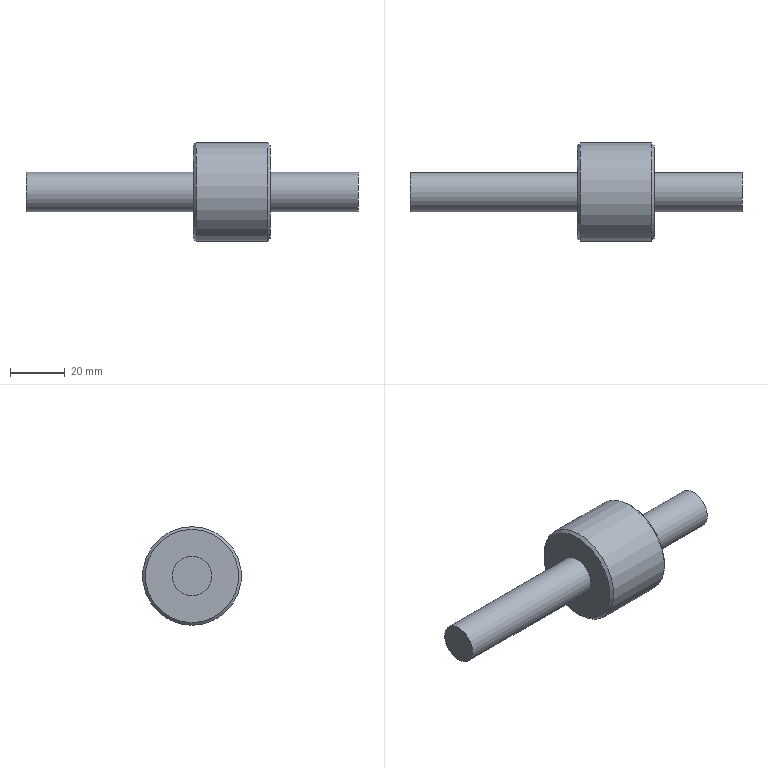Component | NX | 36_LOCATING_PIN | 1 solid | 9 faces | box 121 x 36 x 36 mm | volume 43485 mm3 | plane 4 | cylinder 3 | cone 2 | commonest cylinder face diameters 14.376 x2 36 x1
STEP:
#1=CARTESIAN_POINT('',(0.,0.,0.));
#2=DIRECTION('',(0.,0.,1.));
#3=DIRECTION('',(1.,0.,0.));
#4=AXIS2_PLACEMENT_3D('',#1,#2,#3);
#5=CARTESIAN_POINT('',(45.,40.,-18.));
#6=VERTEX_POINT('',#5);
#7=CARTESIAN_POINT('',(45.,40.,-0.));
#8=DIRECTION('',(-1.,0.,0.));
#9=DIRECTION('',(0.,0.,-1.));
#10=AXIS2_PLACEMENT_3D('',#7,#8,#9);
#11=CIRCLE('',#10,18.);
#12=CARTESIAN_POINT('',(46.,40.,-0.));
#13=DIRECTION('',(-1.,0.,0.));
#14=DIRECTION('',(0.,0.,1.));
#15=AXIS2_PLACEMENT_3D('',#12,#13,#14);
#16=CYLINDRICAL_SURFACE('',#15,18.);
#17=CARTESIAN_POINT('',(3.142,1.));
#18=DIRECTION('',(1.,0.));
#19=VECTOR('',#18,1.);
#20=LINE('',#17,#19);
#21=(GEOMETRIC_REPRESENTATION_CONTEXT(2)PARAMETRIC_REPRESENTATION_CONTEXT()REPRESENTATION_CONTEXT('',''));
#22=DEFINITIONAL_REPRESENTATION('',(#20),#21);
#23=PCURVE('',#16,#22);
#24=CARTESIAN_POINT('',(46.,40.,-0.));
#25=DIRECTION('',(-1.,0.,0.));
#26=DIRECTION('',(0.,0.,1.));
#27=AXIS2_PLACEMENT_3D('',#24,#25,#26);
#28=CONICAL_SURFACE('',#27,17.,0.7854);
#29=CARTESIAN_POINT('',(3.142,1.));
#30=DIRECTION('',(1.,0.));
#31=VECTOR('',#30,1.);
#32=LINE('',#29,#31);
#33=(GEOMETRIC_REPRESENTATION_CONTEXT(2)PARAMETRIC_REPRESENTATION_CONTEXT()REPRESENTATION_CONTEXT('',''));
#34=DEFINITIONAL_REPRESENTATION('',(#32),#33);
#35=PCURVE('',#28,#34);
#36=SURFACE_CURVE('',#11,(#23,#35),.PCURVE_S1.);
#37=EDGE_CURVE('',#6,#6,#36,.T.);
#38=ORIENTED_EDGE('',*,*,#37,.T.);
#39=CARTESIAN_POINT('',(19.,40.,-18.));
#40=VERTEX_POINT('',#39);
#41=CARTESIAN_POINT('',(45.,40.,-18.));
#42=CARTESIAN_POINT('',(19.,40.,-18.));
#43=B_SPLINE_CURVE_WITH_KNOTS('',1,(#41,#42),.UNSPECIFIED.,.F.,.F.,(2,2),(1.,27.),.PIECEWISE_BEZIER_KNOTS.);
#44=CARTESIAN_POINT('',(9.425,0.));
#45=DIRECTION('',(0.,1.));
#46=VECTOR('',#45,1.);
#47=LINE('',#44,#46);
#48=(GEOMETRIC_REPRESENTATION_CONTEXT(2)PARAMETRIC_REPRESENTATION_CONTEXT()REPRESENTATION_CONTEXT('',''));
#49=DEFINITIONAL_REPRESENTATION('',(#47),#48);
#50=PCURVE('',#16,#49);
#51=CARTESIAN_POINT('',(3.142,0.));
#52=DIRECTION('',(0.,1.));
#53=VECTOR('',#52,1.);
#54=LINE('',#51,#53);
#55=(GEOMETRIC_REPRESENTATION_CONTEXT(2)PARAMETRIC_REPRESENTATION_CONTEXT()REPRESENTATION_CONTEXT('',''));
#56=DEFINITIONAL_REPRESENTATION('',(#54),#55);
#57=PCURVE('',#16,#56);
#58=SEAM_CURVE('',#43,(#50,#57),.PCURVE_S1.);
#59=EDGE_CURVE('',#6,#40,#58,.T.);
#60=ORIENTED_EDGE('',*,*,#59,.T.);
#61=CARTESIAN_POINT('',(19.,40.,-0.));
#62=DIRECTION('',(1.,0.,0.));
#63=DIRECTION('',(0.,0.,-1.));
#64=AXIS2_PLACEMENT_3D('',#61,#62,#63);
#65=CIRCLE('',#64,18.);
#66=CARTESIAN_POINT('',(9.425,27.));
#67=DIRECTION('',(-1.,0.));
#68=VECTOR('',#67,1.);
#69=LINE('',#66,#68);
#70=(GEOMETRIC_REPRESENTATION_CONTEXT(2)PARAMETRIC_REPRESENTATION_CONTEXT()REPRESENTATION_CONTEXT('',''));
#71=DEFINITIONAL_REPRESENTATION('',(#69),#70);
#72=PCURVE('',#16,#71);
#73=CARTESIAN_POINT('',(19.,40.,-0.));
#74=DIRECTION('',(1.,0.,0.));
#75=DIRECTION('',(0.,0.,-1.));
#76=AXIS2_PLACEMENT_3D('',#73,#74,#75);
#77=CONICAL_SURFACE('',#76,18.,0.7854);
#78=CARTESIAN_POINT('',(0.,0.));
#79=DIRECTION('',(1.,0.));
#80=VECTOR('',#79,1.);
#81=LINE('',#78,#80);
#82=(GEOMETRIC_REPRESENTATION_CONTEXT(2)PARAMETRIC_REPRESENTATION_CONTEXT()REPRESENTATION_CONTEXT('',''));
#83=DEFINITIONAL_REPRESENTATION('',(#81),#82);
#84=PCURVE('',#77,#83);
#85=SURFACE_CURVE('',#65,(#72,#84),.PCURVE_S1.);
#86=EDGE_CURVE('',#40,#40,#85,.T.);
#87=ORIENTED_EDGE('',*,*,#86,.T.);
#88=ORIENTED_EDGE('',*,*,#59,.F.);
#89=EDGE_LOOP('',(#38,#60,#87,#88));
#90=FACE_BOUND('',#89,.T.);
#91=ADVANCED_FACE('',(#90),#16,.T.);
#92=CARTESIAN_POINT('',(46.,40.,-17.));
#93=VERTEX_POINT('',#92);
#94=CARTESIAN_POINT('',(46.,40.,-0.));
#95=DIRECTION('',(1.,0.,0.));
#96=DIRECTION('',(0.,0.,-1.));
#97=AXIS2_PLACEMENT_3D('',#94,#95,#96);
#98=CIRCLE('',#97,17.);
#99=CARTESIAN_POINT('',(46.,40.,-0.));
#100=DIRECTION('',(1.,0.,0.));
#101=DIRECTION('',(0.,0.,-1.));
#102=AXIS2_PLACEMENT_3D('',#99,#100,#101);
#103=PLANE('',#102);
#104=CARTESIAN_POINT('',(0.,0.));
#105=DIRECTION('',(1.,0.));
#106=AXIS2_PLACEMENT_2D('',#104,#105);
#107=CIRCLE('',#106,17.);
#108=(GEOMETRIC_REPRESENTATION_CONTEXT(2)PARAMETRIC_REPRESENTATION_CONTEXT()REPRESENTATION_CONTEXT('',''));
#109=DEFINITIONAL_REPRESENTATION('',(#107),#108);
#110=PCURVE('',#103,#109);
#111=CARTESIAN_POINT('',(9.425,0.));
#112=DIRECTION('',(-1.,0.));
#113=VECTOR('',#112,1.);
#114=LINE('',#111,#113);
#115=(GEOMETRIC_REPRESENTATION_CONTEXT(2)PARAMETRIC_REPRESENTATION_CONTEXT()REPRESENTATION_CONTEXT('',''));
#116=DEFINITIONAL_REPRESENTATION('',(#114),#115);
#117=PCURVE('',#28,#116);
#118=SURFACE_CURVE('',#98,(#110,#117),.PCURVE_S1.);
#119=EDGE_CURVE('',#93,#93,#118,.T.);
#120=ORIENTED_EDGE('',*,*,#119,.T.);
#121=EDGE_LOOP('',(#120));
#122=FACE_BOUND('',#121,.T.);
#123=CARTESIAN_POINT('',(46.,40.,-7.188));
#124=VERTEX_POINT('',#123);
#125=CARTESIAN_POINT('',(46.,40.,-0.));
#126=DIRECTION('',(-1.,0.,0.));
#127=DIRECTION('',(0.,0.,-1.));
#128=AXIS2_PLACEMENT_3D('',#125,#126,#127);
#129=CIRCLE('',#128,7.188);
#130=CARTESIAN_POINT('',(7.188,0.));
#131=CARTESIAN_POINT('',(7.188,-12.45));
#132=CARTESIAN_POINT('',(-3.594,-6.225));
#133=CARTESIAN_POINT('',(-14.376,-0.));
#134=CARTESIAN_POINT('',(-3.594,6.225));
#135=CARTESIAN_POINT('',(7.188,12.45));
#136=CARTESIAN_POINT('',(7.188,0.));
#137=(BOUNDED_CURVE()B_SPLINE_CURVE(2,(#130,#131,#132,#133,#134,#135,#136),.UNSPECIFIED.,.T.,.F.)B_SPLINE_CURVE_WITH_KNOTS((1,2,2,2,2,1),(-2.094,0.,2.094,4.189,6.283,8.378),.UNSPECIFIED.)CURVE()GEOMETRIC_REPRESENTATION_ITEM()RATIONAL_B_SPLINE_CURVE((1.,0.5,1.,0.5,1.,0.5,1.))REPRESENTATION_ITEM(''));
#138=(GEOMETRIC_REPRESENTATION_CONTEXT(2)PARAMETRIC_REPRESENTATION_CONTEXT()REPRESENTATION_CONTEXT('',''));
#139=DEFINITIONAL_REPRESENTATION('',(#137),#138);
#140=PCURVE('',#103,#139);
#141=CARTESIAN_POINT('',(78.,40.,-0.));
#142=DIRECTION('',(-1.,0.,0.));
#143=DIRECTION('',(0.,0.,1.));
#144=AXIS2_PLACEMENT_3D('',#141,#142,#143);
#145=CYLINDRICAL_SURFACE('',#144,7.188);
#146=CARTESIAN_POINT('',(3.142,32.));
#147=DIRECTION('',(1.,0.));
#148=VECTOR('',#147,1.);
#149=LINE('',#146,#148);
#150=(GEOMETRIC_REPRESENTATION_CONTEXT(2)PARAMETRIC_REPRESENTATION_CONTEXT()REPRESENTATION_CONTEXT('',''));
#151=DEFINITIONAL_REPRESENTATION('',(#149),#150);
#152=PCURVE('',#145,#151);
#153=SURFACE_CURVE('',#129,(#140,#152),.PCURVE_S1.);
#154=EDGE_CURVE('',#124,#124,#153,.T.);
#155=ORIENTED_EDGE('',*,*,#154,.T.);
#156=EDGE_LOOP('',(#155));
#157=FACE_BOUND('',#156,.T.);
#158=ADVANCED_FACE('',(#122,#157),#103,.T.);
#159=CARTESIAN_POINT('',(18.,40.,-17.));
#160=VERTEX_POINT('',#159);
#161=CARTESIAN_POINT('',(18.,40.,-0.));
#162=DIRECTION('',(-1.,0.,0.));
#163=DIRECTION('',(0.,0.,-1.));
#164=AXIS2_PLACEMENT_3D('',#161,#162,#163);
#165=CIRCLE('',#164,17.);
#166=CARTESIAN_POINT('',(18.,40.,-0.));
#167=DIRECTION('',(1.,0.,0.));
#168=DIRECTION('',(0.,0.,-1.));
#169=AXIS2_PLACEMENT_3D('',#166,#167,#168);
#170=PLANE('',#169);
#171=CARTESIAN_POINT('',(17.,0.));
#172=CARTESIAN_POINT('',(17.,-29.445));
#173=CARTESIAN_POINT('',(-8.5,-14.722));
#174=CARTESIAN_POINT('',(-34.,-0.));
#175=CARTESIAN_POINT('',(-8.5,14.722));
#176=CARTESIAN_POINT('',(17.,29.445));
#177=CARTESIAN_POINT('',(17.,0.));
#178=(BOUNDED_CURVE()B_SPLINE_CURVE(2,(#171,#172,#173,#174,#175,#176,#177),.UNSPECIFIED.,.T.,.F.)B_SPLINE_CURVE_WITH_KNOTS((1,2,2,2,2,1),(-2.094,0.,2.094,4.189,6.283,8.378),.UNSPECIFIED.)CURVE()GEOMETRIC_REPRESENTATION_ITEM()RATIONAL_B_SPLINE_CURVE((1.,0.5,1.,0.5,1.,0.5,1.))REPRESENTATION_ITEM(''));
#179=(GEOMETRIC_REPRESENTATION_CONTEXT(2)PARAMETRIC_REPRESENTATION_CONTEXT()REPRESENTATION_CONTEXT('',''));
#180=DEFINITIONAL_REPRESENTATION('',(#178),#179);
#181=PCURVE('',#170,#180);
#182=CARTESIAN_POINT('',(6.283,-1.));
#183=DIRECTION('',(-1.,0.));
#184=VECTOR('',#183,1.);
#185=LINE('',#182,#184);
#186=(GEOMETRIC_REPRESENTATION_CONTEXT(2)PARAMETRIC_REPRESENTATION_CONTEXT()REPRESENTATION_CONTEXT('',''));
#187=DEFINITIONAL_REPRESENTATION('',(#185),#186);
#188=PCURVE('',#77,#187);
#189=SURFACE_CURVE('',#165,(#181,#188),.PCURVE_S1.);
#190=EDGE_CURVE('',#160,#160,#189,.T.);
#191=ORIENTED_EDGE('',*,*,#190,.T.);
#192=EDGE_LOOP('',(#191));
#193=FACE_BOUND('',#192,.T.);
#194=CARTESIAN_POINT('',(18.,40.,-7.188));
#195=VERTEX_POINT('',#194);
#196=CARTESIAN_POINT('',(18.,40.,-0.));
#197=DIRECTION('',(-1.,0.,0.));
#198=DIRECTION('',(0.,0.,-1.));
#199=AXIS2_PLACEMENT_3D('',#196,#197,#198);
#200=CIRCLE('',#199,7.188);
#201=CARTESIAN_POINT('',(7.188,0.));
#202=CARTESIAN_POINT('',(7.188,-12.45));
#203=CARTESIAN_POINT('',(-3.594,-6.225));
#204=CARTESIAN_POINT('',(-14.376,-0.));
#205=CARTESIAN_POINT('',(-3.594,6.225));
#206=CARTESIAN_POINT('',(7.188,12.45));
#207=CARTESIAN_POINT('',(7.188,0.));
#208=(BOUNDED_CURVE()B_SPLINE_CURVE(2,(#201,#202,#203,#204,#205,#206,#207),.UNSPECIFIED.,.T.,.F.)B_SPLINE_CURVE_WITH_KNOTS((1,2,2,2,2,1),(-2.094,0.,2.094,4.189,6.283,8.378),.UNSPECIFIED.)CURVE()GEOMETRIC_REPRESENTATION_ITEM()RATIONAL_B_SPLINE_CURVE((1.,0.5,1.,0.5,1.,0.5,1.))REPRESENTATION_ITEM(''));
#209=(GEOMETRIC_REPRESENTATION_CONTEXT(2)PARAMETRIC_REPRESENTATION_CONTEXT()REPRESENTATION_CONTEXT('',''));
#210=DEFINITIONAL_REPRESENTATION('',(#208),#209);
#211=PCURVE('',#170,#210);
#212=CARTESIAN_POINT('',(78.,40.,-0.));
#213=DIRECTION('',(-1.,0.,0.));
#214=DIRECTION('',(0.,0.,1.));
#215=AXIS2_PLACEMENT_3D('',#212,#213,#214);
#216=CYLINDRICAL_SURFACE('',#215,7.188);
#217=CARTESIAN_POINT('',(3.142,60.));
#218=DIRECTION('',(1.,0.));
#219=VECTOR('',#218,1.);
#220=LINE('',#217,#219);
#221=(GEOMETRIC_REPRESENTATION_CONTEXT(2)PARAMETRIC_REPRESENTATION_CONTEXT()REPRESENTATION_CONTEXT('',''));
#222=DEFINITIONAL_REPRESENTATION('',(#220),#221);
#223=PCURVE('',#216,#222);
#224=SURFACE_CURVE('',#200,(#211,#223),.PCURVE_S1.);
#225=EDGE_CURVE('',#195,#195,#224,.T.);
#226=ORIENTED_EDGE('',*,*,#225,.F.);
#227=EDGE_LOOP('',(#226));
#228=FACE_BOUND('',#227,.T.);
#229=ADVANCED_FACE('',(#193,#228),#170,.F.);
#230=CARTESIAN_POINT('',(-43.,40.,-7.188));
#231=VERTEX_POINT('',#230);
#232=CARTESIAN_POINT('',(-43.,40.,-0.));
#233=DIRECTION('',(1.,0.,0.));
#234=DIRECTION('',(0.,0.,-1.));
#235=AXIS2_PLACEMENT_3D('',#232,#233,#234);
#236=CIRCLE('',#235,7.188);
#237=CARTESIAN_POINT('',(-43.,40.,-0.));
#238=DIRECTION('',(1.,0.,0.));
#239=DIRECTION('',(0.,0.,-1.));
#240=AXIS2_PLACEMENT_3D('',#237,#238,#239);
#241=PLANE('',#240);
#242=CARTESIAN_POINT('',(0.,0.));
#243=DIRECTION('',(1.,0.));
#244=AXIS2_PLACEMENT_2D('',#242,#243);
#245=CIRCLE('',#244,7.188);
#246=(GEOMETRIC_REPRESENTATION_CONTEXT(2)PARAMETRIC_REPRESENTATION_CONTEXT()REPRESENTATION_CONTEXT('',''));
#247=DEFINITIONAL_REPRESENTATION('',(#245),#246);
#248=PCURVE('',#241,#247);
#249=CARTESIAN_POINT('',(9.425,121.));
#250=DIRECTION('',(-1.,0.));
#251=VECTOR('',#250,1.);
#252=LINE('',#249,#251);
#253=(GEOMETRIC_REPRESENTATION_CONTEXT(2)PARAMETRIC_REPRESENTATION_CONTEXT()REPRESENTATION_CONTEXT('',''));
#254=DEFINITIONAL_REPRESENTATION('',(#252),#253);
#255=PCURVE('',#216,#254);
#256=SURFACE_CURVE('',#236,(#248,#255),.PCURVE_S1.);
#257=EDGE_CURVE('',#231,#231,#256,.T.);
#258=ORIENTED_EDGE('',*,*,#257,.F.);
#259=EDGE_LOOP('',(#258));
#260=FACE_BOUND('',#259,.T.);
#261=ADVANCED_FACE('',(#260),#241,.F.);
#262=ORIENTED_EDGE('',*,*,#257,.T.);
#263=CARTESIAN_POINT('',(18.,40.,-7.188));
#264=CARTESIAN_POINT('',(-43.,40.,-7.188));
#265=B_SPLINE_CURVE_WITH_KNOTS('',1,(#263,#264),.UNSPECIFIED.,.F.,.F.,(2,2),(60.,121.),.PIECEWISE_BEZIER_KNOTS.);
#266=CARTESIAN_POINT('',(3.142,0.));
#267=DIRECTION('',(0.,1.));
#268=VECTOR('',#267,1.);
#269=LINE('',#266,#268);
#270=(GEOMETRIC_REPRESENTATION_CONTEXT(2)PARAMETRIC_REPRESENTATION_CONTEXT()REPRESENTATION_CONTEXT('',''));
#271=DEFINITIONAL_REPRESENTATION('',(#269),#270);
#272=PCURVE('',#216,#271);
#273=CARTESIAN_POINT('',(9.425,0.));
#274=DIRECTION('',(0.,1.));
#275=VECTOR('',#274,1.);
#276=LINE('',#273,#275);
#277=(GEOMETRIC_REPRESENTATION_CONTEXT(2)PARAMETRIC_REPRESENTATION_CONTEXT()REPRESENTATION_CONTEXT('',''));
#278=DEFINITIONAL_REPRESENTATION('',(#276),#277);
#279=PCURVE('',#216,#278);
#280=SEAM_CURVE('',#265,(#272,#279),.PCURVE_S1.);
#281=EDGE_CURVE('',#195,#231,#280,.T.);
#282=ORIENTED_EDGE('',*,*,#281,.F.);
#283=ORIENTED_EDGE('',*,*,#225,.T.);
#284=ORIENTED_EDGE('',*,*,#281,.T.);
#285=EDGE_LOOP('',(#262,#282,#283,#284));
#286=FACE_BOUND('',#285,.T.);
#287=ADVANCED_FACE('',(#286),#216,.T.);
#288=ORIENTED_EDGE('',*,*,#154,.F.);
#289=CARTESIAN_POINT('',(78.,40.,-7.188));
#290=VERTEX_POINT('',#289);
#291=CARTESIAN_POINT('',(78.,40.,-7.188));
#292=CARTESIAN_POINT('',(46.,40.,-7.188));
#293=B_SPLINE_CURVE_WITH_KNOTS('',1,(#291,#292),.UNSPECIFIED.,.F.,.F.,(2,2),(0.,32.),.PIECEWISE_BEZIER_KNOTS.);
#294=CARTESIAN_POINT('',(3.142,0.));
#295=DIRECTION('',(0.,1.));
#296=VECTOR('',#295,1.);
#297=LINE('',#294,#296);
#298=(GEOMETRIC_REPRESENTATION_CONTEXT(2)PARAMETRIC_REPRESENTATION_CONTEXT()REPRESENTATION_CONTEXT('',''));
#299=DEFINITIONAL_REPRESENTATION('',(#297),#298);
#300=PCURVE('',#145,#299);
#301=CARTESIAN_POINT('',(9.425,0.));
#302=DIRECTION('',(0.,1.));
#303=VECTOR('',#302,1.);
#304=LINE('',#301,#303);
#305=(GEOMETRIC_REPRESENTATION_CONTEXT(2)PARAMETRIC_REPRESENTATION_CONTEXT()REPRESENTATION_CONTEXT('',''));
#306=DEFINITIONAL_REPRESENTATION('',(#304),#305);
#307=PCURVE('',#145,#306);
#308=SEAM_CURVE('',#293,(#300,#307),.PCURVE_S1.);
#309=EDGE_CURVE('',#290,#124,#308,.T.);
#310=ORIENTED_EDGE('',*,*,#309,.F.);
#311=CARTESIAN_POINT('',(78.,40.,-0.));
#312=DIRECTION('',(1.,0.,0.));
#313=DIRECTION('',(0.,0.,-1.));
#314=AXIS2_PLACEMENT_3D('',#311,#312,#313);
#315=CIRCLE('',#314,7.188);
#316=CARTESIAN_POINT('',(9.425,0.));
#317=DIRECTION('',(-1.,0.));
#318=VECTOR('',#317,1.);
#319=LINE('',#316,#318);
#320=(GEOMETRIC_REPRESENTATION_CONTEXT(2)PARAMETRIC_REPRESENTATION_CONTEXT()REPRESENTATION_CONTEXT('',''));
#321=DEFINITIONAL_REPRESENTATION('',(#319),#320);
#322=PCURVE('',#145,#321);
#323=CARTESIAN_POINT('',(78.,40.,-0.));
#324=DIRECTION('',(1.,0.,0.));
#325=DIRECTION('',(0.,0.,-1.));
#326=AXIS2_PLACEMENT_3D('',#323,#324,#325);
#327=PLANE('',#326);
#328=CARTESIAN_POINT('',(0.,0.));
#329=DIRECTION('',(1.,0.));
#330=AXIS2_PLACEMENT_2D('',#328,#329);
#331=CIRCLE('',#330,7.188);
#332=(GEOMETRIC_REPRESENTATION_CONTEXT(2)PARAMETRIC_REPRESENTATION_CONTEXT()REPRESENTATION_CONTEXT('',''));
#333=DEFINITIONAL_REPRESENTATION('',(#331),#332);
#334=PCURVE('',#327,#333);
#335=SURFACE_CURVE('',#315,(#322,#334),.PCURVE_S1.);
#336=EDGE_CURVE('',#290,#290,#335,.T.);
#337=ORIENTED_EDGE('',*,*,#336,.F.);
#338=ORIENTED_EDGE('',*,*,#309,.T.);
#339=EDGE_LOOP('',(#288,#310,#337,#338));
#340=FACE_BOUND('',#339,.T.);
#341=ADVANCED_FACE('',(#340),#145,.T.);
#342=ORIENTED_EDGE('',*,*,#336,.T.);
#343=EDGE_LOOP('',(#342));
#344=FACE_BOUND('',#343,.T.);
#345=ADVANCED_FACE('',(#344),#327,.T.);
#346=ORIENTED_EDGE('',*,*,#37,.F.);
#347=CARTESIAN_POINT('',(46.,40.,-17.));
#348=CARTESIAN_POINT('',(45.,40.,-18.));
#349=B_SPLINE_CURVE_WITH_KNOTS('',1,(#347,#348),.UNSPECIFIED.,.F.,.F.,(2,2),(0.,1.414),.PIECEWISE_BEZIER_KNOTS.);
#350=CARTESIAN_POINT('',(3.142,0.));
#351=DIRECTION('',(0.,1.));
#352=VECTOR('',#351,1.);
#353=LINE('',#350,#352);
#354=(GEOMETRIC_REPRESENTATION_CONTEXT(2)PARAMETRIC_REPRESENTATION_CONTEXT()REPRESENTATION_CONTEXT('',''));
#355=DEFINITIONAL_REPRESENTATION('',(#353),#354);
#356=PCURVE('',#28,#355);
#357=CARTESIAN_POINT('',(9.425,0.));
#358=DIRECTION('',(0.,1.));
#359=VECTOR('',#358,1.);
#360=LINE('',#357,#359);
#361=(GEOMETRIC_REPRESENTATION_CONTEXT(2)PARAMETRIC_REPRESENTATION_CONTEXT()REPRESENTATION_CONTEXT('',''));
#362=DEFINITIONAL_REPRESENTATION('',(#360),#361);
#363=PCURVE('',#28,#362);
#364=SEAM_CURVE('',#349,(#356,#363),.PCURVE_S1.);
#365=EDGE_CURVE('',#93,#6,#364,.T.);
#366=ORIENTED_EDGE('',*,*,#365,.F.);
#367=ORIENTED_EDGE('',*,*,#119,.F.);
#368=ORIENTED_EDGE('',*,*,#365,.T.);
#369=EDGE_LOOP('',(#346,#366,#367,#368));
#370=FACE_BOUND('',#369,.T.);
#371=ADVANCED_FACE('',(#370),#28,.T.);
#372=ORIENTED_EDGE('',*,*,#190,.F.);
#373=CARTESIAN_POINT('',(18.,40.,-17.));
#374=CARTESIAN_POINT('',(19.,40.,-18.));
#375=B_SPLINE_CURVE_WITH_KNOTS('',1,(#373,#374),.UNSPECIFIED.,.F.,.F.,(2,2),(-1.414,0.),.PIECEWISE_BEZIER_KNOTS.);
#376=CARTESIAN_POINT('',(6.283,0.));
#377=DIRECTION('',(0.,1.));
#378=VECTOR('',#377,1.);
#379=LINE('',#376,#378);
#380=(GEOMETRIC_REPRESENTATION_CONTEXT(2)PARAMETRIC_REPRESENTATION_CONTEXT()REPRESENTATION_CONTEXT('',''));
#381=DEFINITIONAL_REPRESENTATION('',(#379),#380);
#382=PCURVE('',#77,#381);
#383=CARTESIAN_POINT('',(0.,0.));
#384=DIRECTION('',(0.,1.));
#385=VECTOR('',#384,1.);
#386=LINE('',#383,#385);
#387=(GEOMETRIC_REPRESENTATION_CONTEXT(2)PARAMETRIC_REPRESENTATION_CONTEXT()REPRESENTATION_CONTEXT('',''));
#388=DEFINITIONAL_REPRESENTATION('',(#386),#387);
#389=PCURVE('',#77,#388);
#390=SEAM_CURVE('',#375,(#382,#389),.PCURVE_S1.);
#391=EDGE_CURVE('',#160,#40,#390,.T.);
#392=ORIENTED_EDGE('',*,*,#391,.T.);
#393=ORIENTED_EDGE('',*,*,#86,.F.);
#394=ORIENTED_EDGE('',*,*,#391,.F.);
#395=EDGE_LOOP('',(#372,#392,#393,#394));
#396=FACE_BOUND('',#395,.T.);
#397=ADVANCED_FACE('',(#396),#77,.T.);
#398=CLOSED_SHELL('',(#91,#158,#229,#261,#287,#341,#345,#371,#397));
#399=MANIFOLD_SOLID_BREP('',#398);
#400=(LENGTH_UNIT()NAMED_UNIT(*)SI_UNIT(.MILLI.,.METRE.));
#401=UNCERTAINTY_MEASURE_WITH_UNIT(LENGTH_MEASURE(0.00001),#400,'','');
#402=(NAMED_UNIT(*)PLANE_ANGLE_UNIT()SI_UNIT($,.RADIAN.));
#403=(NAMED_UNIT(*)SI_UNIT($,.STERADIAN.)SOLID_ANGLE_UNIT());
#404=(GEOMETRIC_REPRESENTATION_CONTEXT(3)GLOBAL_UNCERTAINTY_ASSIGNED_CONTEXT((#401))GLOBAL_UNIT_ASSIGNED_CONTEXT((#400,#402,#403))REPRESENTATION_CONTEXT('',''));
#405=ADVANCED_BREP_SHAPE_REPRESENTATION('',(#4,#399),#404);